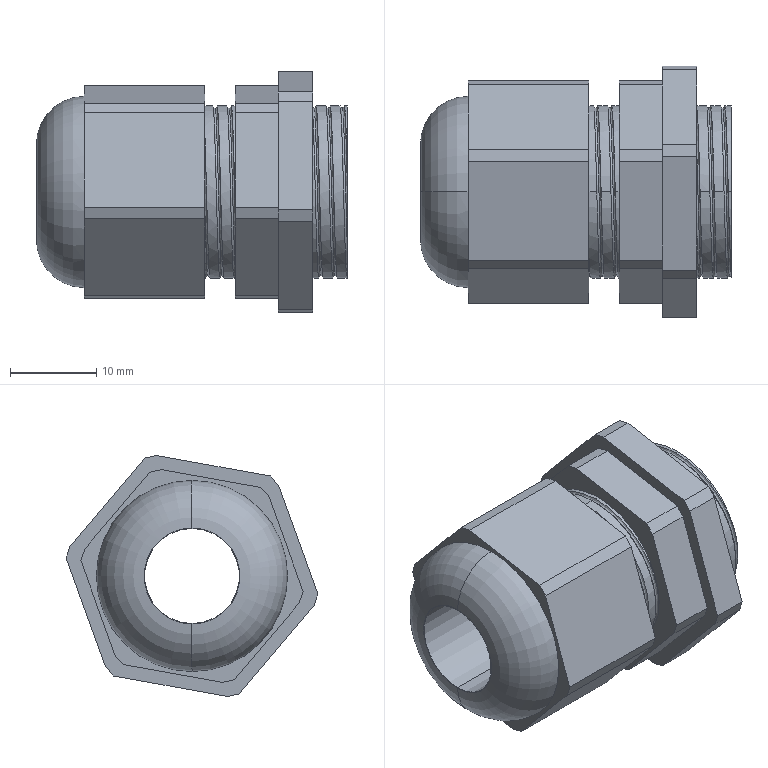Component | SolidWorks | CableGlandPG13.5Black-1 | 1 solid | 65 faces | volume 11630 mm3 | plane 43 | cylinder 16 | spline 4 | torus 2 | commonest cylinder face diameters 20 x14 11 x2